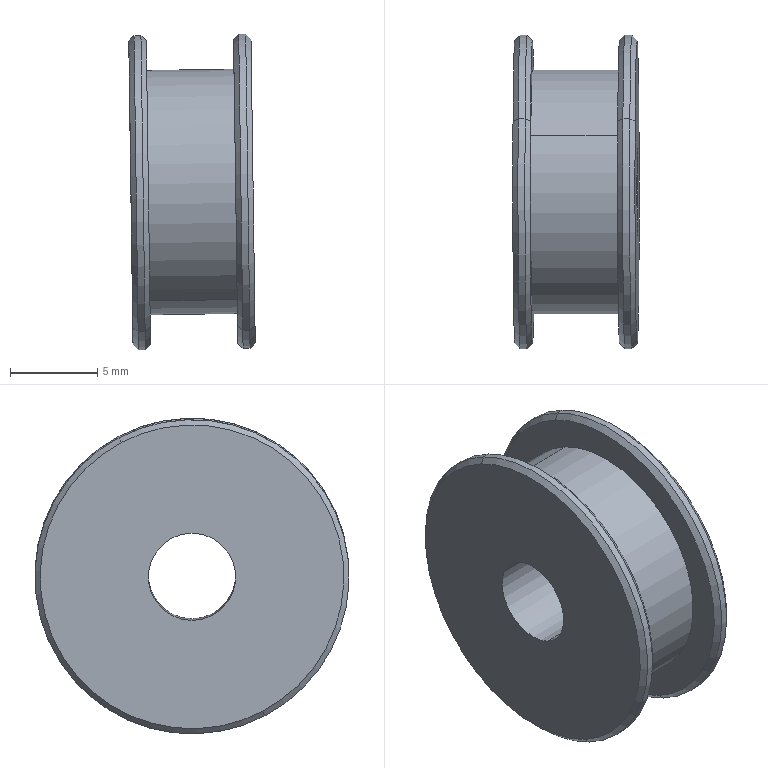Component | SolidWorks | DA-0220-Part11-12 | 1 solid | 20 faces | box 7.24 x 18 x 18.09 mm | volume 1131 mm3 | cone 8 | cylinder 8 | plane 4 | commonest cylinder face diameters 18 x4 14 x2 5 x2
build123d program:
from build123d import *

# Parameters (mm, degrees)
CHAMFER1_SIZE = 0.3


with BuildPart() as part:
    # Sketch1 → Revolve1 (revolve)
    with BuildSketch(Plane.XY, mode=Mode.PRIVATE) as revolve1_sk:
        Polygon((-9, 3.5), (-2.5, 3.5), (-2.5, -3.5), (-9, -3.5), (-9, -2.5), (-7, -2.5), (-7, 2.5), (-9, 2.5), align=None)
    revolve(revolve1_sk.sketch.rotate(Axis((0, 0, 0), (0, -1, 0)), 270), axis=Axis((0, 0, 0), (0, -1, 0)))

    # Chamfer1
    chamfer1_edges = [part.edges().sort_by_distance(p)[0] for p in [
        (0, 2.5, -9),
        (0, -2.5, -9),
        (0, -3.5, -9),
        (0, 3.5, -9),
    ]]
    chamfer(chamfer1_edges, length=CHAMFER1_SIZE)


solid = part.part

# Placed as in the assembly
solid = solid.moved(Location((642.057, -33.791, 552.514), (177.304, 0.7997, 90.014)))
STEP:
#1=COLOUR_RGB('',0.7922,0.8196,0.9333);
#2=FILL_AREA_STYLE_COLOUR('',#1);
#3=FILL_AREA_STYLE('',(#2));
#4=SURFACE_STYLE_FILL_AREA(#3);
#5=SURFACE_SIDE_STYLE('',(#4));
#6=SURFACE_STYLE_USAGE(.BOTH.,#5);
#7=PRESENTATION_STYLE_ASSIGNMENT((#6));
#8=CARTESIAN_POINT('',(25.184,-1.49,21.448));
#9=VERTEX_POINT('',#8);
#10=CARTESIAN_POINT('',(25.175,-1.171,22.054));
#11=VERTEX_POINT('',#10);
#12=CARTESIAN_POINT('',(25.179,-1.33,21.751));
#13=DIRECTION('',(0.9999,0.000404,0.01395));
#14=DIRECTION('',(0.01254,-0.4647,-0.8854));
#15=AXIS2_PLACEMENT_3D('',#12,#13,#14);
#16=CIRCLE('',#15,0.3425);
#17=EDGE_CURVE('',#9,#11,#16,.T.);
#18=ORIENTED_EDGE('',*,*,#17,.F.);
#19=CARTESIAN_POINT('',(25.172,-1.495,21.437));
#20=VERTEX_POINT('',#19);
#21=CARTESIAN_POINT('',(25.172,-1.495,21.437));
#22=DIRECTION('',(-0.6982,-0.3289,-0.6359));
#23=VECTOR('',#22,39.37);
#24=LINE('',#21,#23);
#25=EDGE_CURVE('',#9,#20,#24,.T.);
#26=ORIENTED_EDGE('',*,*,#25,.T.);
#27=CARTESIAN_POINT('',(25.163,-1.166,22.065));
#28=VERTEX_POINT('',#27);
#29=CARTESIAN_POINT('',(25.168,-1.33,21.751));
#30=DIRECTION('',(-0.9999,-0.000404,-0.01395));
#31=DIRECTION('',(0.01254,-0.4647,-0.8854));
#32=AXIS2_PLACEMENT_3D('',#29,#30,#31);
#33=CIRCLE('',#32,0.3543);
#34=EDGE_CURVE('',#28,#20,#33,.T.);
#35=ORIENTED_EDGE('',*,*,#34,.F.);
#36=CARTESIAN_POINT('',(25.163,-1.166,22.065));
#37=DIRECTION('',(-0.7159,0.3283,0.6162));
#38=VECTOR('',#37,39.37);
#39=LINE('',#36,#38);
#40=EDGE_CURVE('',#11,#28,#39,.T.);
#41=ORIENTED_EDGE('',*,*,#40,.F.);
#42=EDGE_LOOP('',(#18,#26,#35,#41));
#43=FACE_OUTER_BOUND('',#42,.T.);
#44=CARTESIAN_POINT('',(25.168,-1.33,21.751));
#45=DIRECTION('',(-0.9999,-0.000404,-0.01395));
#46=DIRECTION('',(-0.01254,0.4647,0.8854));
#47=AXIS2_PLACEMENT_3D('',#44,#45,#46);
#48=CONICAL_SURFACE('',#47,0.3543,0.7854);
#49=ADVANCED_FACE('',(#43),#48,.T.);
#50=CARTESIAN_POINT('',(25.372,-1.171,22.057));
#51=VERTEX_POINT('',#50);
#52=CARTESIAN_POINT('',(25.381,-1.49,21.451));
#53=VERTEX_POINT('',#52);
#54=CARTESIAN_POINT('',(25.376,-1.33,21.754));
#55=DIRECTION('',(-0.9999,-0.000404,-0.01395));
#56=DIRECTION('',(-0.01254,0.4647,0.8854));
#57=AXIS2_PLACEMENT_3D('',#54,#55,#56);
#58=CIRCLE('',#57,0.3425);
#59=EDGE_CURVE('',#51,#53,#58,.T.);
#60=ORIENTED_EDGE('',*,*,#59,.F.);
#61=CARTESIAN_POINT('',(25.384,-1.166,22.068));
#62=VERTEX_POINT('',#61);
#63=CARTESIAN_POINT('',(25.372,-1.171,22.057));
#64=DIRECTION('',(0.6982,0.3289,0.6359));
#65=VECTOR('',#64,39.37);
#66=LINE('',#63,#65);
#67=EDGE_CURVE('',#51,#62,#66,.T.);
#68=ORIENTED_EDGE('',*,*,#67,.T.);
#69=CARTESIAN_POINT('',(25.393,-1.495,21.44));
#70=VERTEX_POINT('',#69);
#71=CARTESIAN_POINT('',(25.388,-1.33,21.754));
#72=DIRECTION('',(0.9999,0.000404,0.01395));
#73=DIRECTION('',(-0.01254,0.4647,0.8854));
#74=AXIS2_PLACEMENT_3D('',#71,#72,#73);
#75=CIRCLE('',#74,0.3543);
#76=EDGE_CURVE('',#70,#62,#75,.T.);
#77=ORIENTED_EDGE('',*,*,#76,.F.);
#78=CARTESIAN_POINT('',(25.381,-1.49,21.451));
#79=DIRECTION('',(0.7159,-0.3283,-0.6162));
#80=VECTOR('',#79,39.37);
#81=LINE('',#78,#80);
#82=EDGE_CURVE('',#53,#70,#81,.T.);
#83=ORIENTED_EDGE('',*,*,#82,.F.);
#84=EDGE_LOOP('',(#60,#68,#77,#83));
#85=FACE_OUTER_BOUND('',#84,.T.);
#86=CARTESIAN_POINT('',(25.376,-1.33,21.754));
#87=DIRECTION('',(0.9999,0.000404,0.01395));
#88=DIRECTION('',(0.01254,-0.4647,-0.8854));
#89=AXIS2_PLACEMENT_3D('',#86,#87,#88);
#90=CONICAL_SURFACE('',#89,0.3425,0.7854);
#91=ADVANCED_FACE('',(#85),#90,.T.);
#92=CARTESIAN_POINT('',(25.42,-1.489,21.451));
#93=VERTEX_POINT('',#92);
#94=CARTESIAN_POINT('',(25.411,-1.171,22.058));
#95=VERTEX_POINT('',#94);
#96=CARTESIAN_POINT('',(25.416,-1.33,21.754));
#97=DIRECTION('',(0.9999,0.000404,0.01395));
#98=DIRECTION('',(0.01254,-0.4647,-0.8854));
#99=AXIS2_PLACEMENT_3D('',#96,#97,#98);
#100=CIRCLE('',#99,0.3425);
#101=EDGE_CURVE('',#93,#95,#100,.T.);
#102=ORIENTED_EDGE('',*,*,#101,.F.);
#103=CARTESIAN_POINT('',(25.408,-1.495,21.441));
#104=VERTEX_POINT('',#103);
#105=CARTESIAN_POINT('',(25.408,-1.495,21.441));
#106=DIRECTION('',(-0.6982,-0.3289,-0.6359));
#107=VECTOR('',#106,39.37);
#108=LINE('',#105,#107);
#109=EDGE_CURVE('',#93,#104,#108,.T.);
#110=ORIENTED_EDGE('',*,*,#109,.T.);
#111=CARTESIAN_POINT('',(25.399,-1.166,22.068));
#112=VERTEX_POINT('',#111);
#113=CARTESIAN_POINT('',(25.404,-1.33,21.754));
#114=DIRECTION('',(-0.9999,-0.000404,-0.01395));
#115=DIRECTION('',(0.01254,-0.4647,-0.8854));
#116=AXIS2_PLACEMENT_3D('',#113,#114,#115);
#117=CIRCLE('',#116,0.3543);
#118=EDGE_CURVE('',#112,#104,#117,.T.);
#119=ORIENTED_EDGE('',*,*,#118,.F.);
#120=CARTESIAN_POINT('',(25.399,-1.166,22.068));
#121=DIRECTION('',(-0.7159,0.3283,0.6162));
#122=VECTOR('',#121,39.37);
#123=LINE('',#120,#122);
#124=EDGE_CURVE('',#95,#112,#123,.T.);
#125=ORIENTED_EDGE('',*,*,#124,.F.);
#126=EDGE_LOOP('',(#102,#110,#119,#125));
#127=FACE_OUTER_BOUND('',#126,.T.);
#128=CARTESIAN_POINT('',(25.404,-1.33,21.754));
#129=DIRECTION('',(-0.9999,-0.000404,-0.01395));
#130=DIRECTION('',(-0.01254,0.4647,0.8854));
#131=AXIS2_PLACEMENT_3D('',#128,#129,#130);
#132=CONICAL_SURFACE('',#131,0.3543,0.7854);
#133=ADVANCED_FACE('',(#127),#132,.T.);
#134=CARTESIAN_POINT('',(25.136,-1.171,22.054));
#135=VERTEX_POINT('',#134);
#136=CARTESIAN_POINT('',(25.144,-1.49,21.447));
#137=VERTEX_POINT('',#136);
#138=CARTESIAN_POINT('',(25.14,-1.33,21.751));
#139=DIRECTION('',(-0.9999,-0.000404,-0.01395));
#140=DIRECTION('',(-0.01254,0.4647,0.8854));
#141=AXIS2_PLACEMENT_3D('',#138,#139,#140);
#142=CIRCLE('',#141,0.3425);
#143=EDGE_CURVE('',#135,#137,#142,.T.);
#144=ORIENTED_EDGE('',*,*,#143,.F.);
#145=CARTESIAN_POINT('',(25.147,-1.166,22.064));
#146=VERTEX_POINT('',#145);
#147=CARTESIAN_POINT('',(25.136,-1.171,22.054));
#148=DIRECTION('',(0.6982,0.3289,0.6359));
#149=VECTOR('',#148,39.37);
#150=LINE('',#147,#149);
#151=EDGE_CURVE('',#135,#146,#150,.T.);
#152=ORIENTED_EDGE('',*,*,#151,.T.);
#153=CARTESIAN_POINT('',(25.156,-1.495,21.437));
#154=VERTEX_POINT('',#153);
#155=CARTESIAN_POINT('',(25.152,-1.33,21.751));
#156=DIRECTION('',(0.9999,0.000404,0.01395));
#157=DIRECTION('',(-0.01254,0.4647,0.8854));
#158=AXIS2_PLACEMENT_3D('',#155,#156,#157);
#159=CIRCLE('',#158,0.3543);
#160=EDGE_CURVE('',#154,#146,#159,.T.);
#161=ORIENTED_EDGE('',*,*,#160,.F.);
#162=CARTESIAN_POINT('',(25.144,-1.49,21.447));
#163=DIRECTION('',(0.7159,-0.3283,-0.6162));
#164=VECTOR('',#163,39.37);
#165=LINE('',#162,#164);
#166=EDGE_CURVE('',#137,#154,#165,.T.);
#167=ORIENTED_EDGE('',*,*,#166,.F.);
#168=EDGE_LOOP('',(#144,#152,#161,#167));
#169=FACE_OUTER_BOUND('',#168,.T.);
#170=CARTESIAN_POINT('',(25.14,-1.33,21.751));
#171=DIRECTION('',(0.9999,0.000404,0.01395));
#172=DIRECTION('',(0.01254,-0.4647,-0.8854));
#173=AXIS2_PLACEMENT_3D('',#170,#171,#172);
#174=CONICAL_SURFACE('',#173,0.3425,0.7854);
#175=ADVANCED_FACE('',(#169),#174,.T.);
#176=CARTESIAN_POINT('',(25.373,-1.202,21.998));
#177=VERTEX_POINT('',#176);
#178=CARTESIAN_POINT('',(25.38,-1.458,21.51));
#179=VERTEX_POINT('',#178);
#180=CARTESIAN_POINT('',(25.376,-1.33,21.754));
#181=DIRECTION('',(-0.9999,-0.000404,-0.01395));
#182=DIRECTION('',(-0.01254,0.4647,0.8854));
#183=AXIS2_PLACEMENT_3D('',#180,#181,#182);
#184=CIRCLE('',#183,0.2756);
#185=EDGE_CURVE('',#177,#179,#184,.T.);
#186=ORIENTED_EDGE('',*,*,#185,.T.);
#187=CARTESIAN_POINT('',(25.183,-1.458,21.507));
#188=VERTEX_POINT('',#187);
#189=CARTESIAN_POINT('',(25.281,-1.458,21.509));
#190=DIRECTION('',(-0.9999,-0.000404,-0.01395));
#191=VECTOR('',#190,39.37);
#192=LINE('',#189,#191);
#193=EDGE_CURVE('',#179,#188,#192,.T.);
#194=ORIENTED_EDGE('',*,*,#193,.T.);
#195=CARTESIAN_POINT('',(25.176,-1.202,21.995));
#196=VERTEX_POINT('',#195);
#197=CARTESIAN_POINT('',(25.179,-1.33,21.751));
#198=DIRECTION('',(-0.9999,-0.000404,-0.01395));
#199=DIRECTION('',(-0.01254,0.4647,0.8854));
#200=AXIS2_PLACEMENT_3D('',#197,#198,#199);
#201=CIRCLE('',#200,0.2756);
#202=EDGE_CURVE('',#196,#188,#201,.T.);
#203=ORIENTED_EDGE('',*,*,#202,.F.);
#204=CARTESIAN_POINT('',(25.274,-1.202,21.997));
#205=DIRECTION('',(-0.9999,-0.000404,-0.01395));
#206=VECTOR('',#205,39.37);
#207=LINE('',#204,#206);
#208=EDGE_CURVE('',#177,#196,#207,.T.);
#209=ORIENTED_EDGE('',*,*,#208,.F.);
#210=EDGE_LOOP('',(#186,#194,#203,#209));
#211=FACE_OUTER_BOUND('',#210,.T.);
#212=CARTESIAN_POINT('',(25.278,-1.33,21.753));
#213=DIRECTION('',(-0.9999,-0.000404,-0.01395));
#214=DIRECTION('',(-0.01254,0.4647,0.8854));
#215=AXIS2_PLACEMENT_3D('',#212,#213,#214);
#216=CYLINDRICAL_SURFACE('',#215,0.2756);
#217=ADVANCED_FACE('',(#211),#216,.T.);
#218=ORIENTED_EDGE('',*,*,#118,.T.);
#219=CARTESIAN_POINT('',(25.282,-1.495,21.439));
#220=DIRECTION('',(-0.9999,-0.000404,-0.01395));
#221=VECTOR('',#220,39.37);
#222=LINE('',#219,#221);
#223=EDGE_CURVE('',#104,#70,#222,.T.);
#224=ORIENTED_EDGE('',*,*,#223,.T.);
#225=ORIENTED_EDGE('',*,*,#76,.T.);
#226=CARTESIAN_POINT('',(25.273,-1.166,22.066));
#227=DIRECTION('',(-0.9999,-0.000404,-0.01395));
#228=VECTOR('',#227,39.37);
#229=LINE('',#226,#228);
#230=EDGE_CURVE('',#112,#62,#229,.T.);
#231=ORIENTED_EDGE('',*,*,#230,.F.);
#232=EDGE_LOOP('',(#218,#224,#225,#231));
#233=FACE_OUTER_BOUND('',#232,.T.);
#234=CARTESIAN_POINT('',(25.278,-1.33,21.753));
#235=DIRECTION('',(-0.9999,-0.000404,-0.01395));
#236=DIRECTION('',(-0.01254,0.4647,0.8854));
#237=AXIS2_PLACEMENT_3D('',#234,#235,#236);
#238=CYLINDRICAL_SURFACE('',#237,0.3543);
#239=ADVANCED_FACE('',(#233),#238,.T.);
#240=CARTESIAN_POINT('',(25.417,-1.376,21.667));
#241=VERTEX_POINT('',#240);
#242=CARTESIAN_POINT('',(25.414,-1.285,21.842));
#243=VERTEX_POINT('',#242);
#244=CARTESIAN_POINT('',(25.416,-1.33,21.754));
#245=DIRECTION('',(-0.9999,-0.000404,-0.01395));
#246=DIRECTION('',(-0.01254,0.4647,0.8854));
#247=AXIS2_PLACEMENT_3D('',#244,#245,#246);
#248=CIRCLE('',#247,0.09843);
#249=EDGE_CURVE('',#241,#243,#248,.T.);
#250=ORIENTED_EDGE('',*,*,#249,.F.);
#251=CARTESIAN_POINT('',(25.141,-1.376,21.663));
#252=VERTEX_POINT('',#251);
#253=CARTESIAN_POINT('',(25.279,-1.376,21.665));
#254=DIRECTION('',(-0.9999,-0.000404,-0.01395));
#255=VECTOR('',#254,39.37);
#256=LINE('',#253,#255);
#257=EDGE_CURVE('',#241,#252,#256,.T.);
#258=ORIENTED_EDGE('',*,*,#257,.T.);
#259=CARTESIAN_POINT('',(25.139,-1.285,21.838));
#260=VERTEX_POINT('',#259);
#261=CARTESIAN_POINT('',(25.14,-1.33,21.751));
#262=DIRECTION('',(-0.9999,-0.000404,-0.01395));
#263=DIRECTION('',(-0.01254,0.4647,0.8854));
#264=AXIS2_PLACEMENT_3D('',#261,#262,#263);
#265=CIRCLE('',#264,0.09843);
#266=EDGE_CURVE('',#252,#260,#265,.T.);
#267=ORIENTED_EDGE('',*,*,#266,.T.);
#268=CARTESIAN_POINT('',(25.277,-1.285,21.84));
#269=DIRECTION('',(-0.9999,-0.000404,-0.01395));
#270=VECTOR('',#269,39.37);
#271=LINE('',#268,#270);
#272=EDGE_CURVE('',#243,#260,#271,.T.);
#273=ORIENTED_EDGE('',*,*,#272,.F.);
#274=EDGE_LOOP('',(#250,#258,#267,#273));
#275=FACE_OUTER_BOUND('',#274,.T.);
#276=CARTESIAN_POINT('',(25.278,-1.33,21.753));
#277=DIRECTION('',(-0.9999,-0.000404,-0.01395));
#278=DIRECTION('',(-0.01254,0.4647,0.8854));
#279=AXIS2_PLACEMENT_3D('',#276,#277,#278);
#280=CYLINDRICAL_SURFACE('',#279,0.09843);
#281=ADVANCED_FACE('',(#275),#280,.F.);
#282=ORIENTED_EDGE('',*,*,#34,.T.);
#283=CARTESIAN_POINT('',(25.282,-1.495,21.439));
#284=DIRECTION('',(-0.9999,-0.000404,-0.01395));
#285=VECTOR('',#284,39.37);
#286=LINE('',#283,#285);
#287=EDGE_CURVE('',#20,#154,#286,.T.);
#288=ORIENTED_EDGE('',*,*,#287,.T.);
#289=ORIENTED_EDGE('',*,*,#160,.T.);
#290=CARTESIAN_POINT('',(25.273,-1.166,22.066));
#291=DIRECTION('',(-0.9999,-0.000404,-0.01395));
#292=VECTOR('',#291,39.37);
#293=LINE('',#290,#292);
#294=EDGE_CURVE('',#28,#146,#293,.T.);
#295=ORIENTED_EDGE('',*,*,#294,.F.);
#296=EDGE_LOOP('',(#282,#288,#289,#295));
#297=FACE_OUTER_BOUND('',#296,.T.);
#298=CARTESIAN_POINT('',(25.278,-1.33,21.753));
#299=DIRECTION('',(-0.9999,-0.000404,-0.01395));
#300=DIRECTION('',(-0.01254,0.4647,0.8854));
#301=AXIS2_PLACEMENT_3D('',#298,#299,#300);
#302=CYLINDRICAL_SURFACE('',#301,0.3543);
#303=ADVANCED_FACE('',(#297),#302,.T.);
#304=ORIENTED_EDGE('',*,*,#287,.F.);
#305=CARTESIAN_POINT('',(25.168,-1.33,21.751));
#306=DIRECTION('',(-0.9999,-0.000404,-0.01395));
#307=DIRECTION('',(0.01254,-0.4647,-0.8854));
#308=AXIS2_PLACEMENT_3D('',#305,#306,#307);
#309=CIRCLE('',#308,0.3543);
#310=EDGE_CURVE('',#20,#28,#309,.T.);
#311=ORIENTED_EDGE('',*,*,#310,.T.);
#312=ORIENTED_EDGE('',*,*,#294,.T.);
#313=CARTESIAN_POINT('',(25.152,-1.33,21.751));
#314=DIRECTION('',(0.9999,0.000404,0.01395));
#315=DIRECTION('',(-0.01254,0.4647,0.8854));
#316=AXIS2_PLACEMENT_3D('',#313,#314,#315);
#317=CIRCLE('',#316,0.3543);
#318=EDGE_CURVE('',#146,#154,#317,.T.);
#319=ORIENTED_EDGE('',*,*,#318,.T.);
#320=EDGE_LOOP('',(#304,#311,#312,#319));
#321=FACE_OUTER_BOUND('',#320,.T.);
#322=CARTESIAN_POINT('',(25.278,-1.33,21.753));
#323=DIRECTION('',(-0.9999,-0.000404,-0.01395));
#324=DIRECTION('',(-0.01254,0.4647,0.8854));
#325=AXIS2_PLACEMENT_3D('',#322,#323,#324);
#326=CYLINDRICAL_SURFACE('',#325,0.3543);
#327=ADVANCED_FACE('',(#321),#326,.T.);
#328=CARTESIAN_POINT('',(25.14,-1.33,21.751));
#329=DIRECTION('',(-0.9999,-0.000404,-0.01395));
#330=DIRECTION('',(-0.01254,0.4647,0.8854));
#331=AXIS2_PLACEMENT_3D('',#328,#329,#330);
#332=CIRCLE('',#331,0.3425);
#333=EDGE_CURVE('',#137,#135,#332,.T.);
#334=ORIENTED_EDGE('',*,*,#333,.T.);
#335=ORIENTED_EDGE('',*,*,#143,.T.);
#336=EDGE_LOOP('',(#334,#335));
#337=FACE_OUTER_BOUND('',#336,.T.);
#338=CARTESIAN_POINT('',(25.14,-1.33,21.751));
#339=DIRECTION('',(-0.9999,-0.000404,-0.01395));
#340=DIRECTION('',(-0.01254,0.4647,0.8854));
#341=AXIS2_PLACEMENT_3D('',#338,#339,#340);
#342=CIRCLE('',#341,0.09843);
#343=EDGE_CURVE('',#260,#252,#342,.T.);
#344=ORIENTED_EDGE('',*,*,#343,.F.);
#345=ORIENTED_EDGE('',*,*,#266,.F.);
#346=EDGE_LOOP('',(#344,#345));
#347=FACE_BOUND('',#346,.T.);
#348=CARTESIAN_POINT('',(25.138,-1.644,21.915));
#349=DIRECTION('',(-0.9999,-0.000404,-0.01395));
#350=DIRECTION('',(-0.01254,0.4647,0.8854));
#351=AXIS2_PLACEMENT_3D('',#348,#349,#350);
#352=PLANE('',#351);
#353=ADVANCED_FACE('',(#337,#347),#352,.T.);
#354=ORIENTED_EDGE('',*,*,#257,.F.);
#355=CARTESIAN_POINT('',(25.416,-1.33,21.754));
#356=DIRECTION('',(-0.9999,-0.000404,-0.01395));
#357=DIRECTION('',(-0.01254,0.4647,0.8854));
#358=AXIS2_PLACEMENT_3D('',#355,#356,#357);
#359=CIRCLE('',#358,0.09843);
#360=EDGE_CURVE('',#243,#241,#359,.T.);
#361=ORIENTED_EDGE('',*,*,#360,.F.);
#362=ORIENTED_EDGE('',*,*,#272,.T.);
#363=ORIENTED_EDGE('',*,*,#343,.T.);
#364=EDGE_LOOP('',(#354,#361,#362,#363));
#365=FACE_OUTER_BOUND('',#364,.T.);
#366=CARTESIAN_POINT('',(25.278,-1.33,21.753));
#367=DIRECTION('',(-0.9999,-0.000404,-0.01395));
#368=DIRECTION('',(-0.01254,0.4647,0.8854));
#369=AXIS2_PLACEMENT_3D('',#366,#367,#368);
#370=CYLINDRICAL_SURFACE('',#369,0.09843);
#371=ADVANCED_FACE('',(#365),#370,.F.);
#372=CARTESIAN_POINT('',(25.416,-1.33,21.754));
#373=DIRECTION('',(0.9999,0.000404,0.01395));
#374=DIRECTION('',(0.01254,-0.4647,-0.8854));
#375=AXIS2_PLACEMENT_3D('',#372,#373,#374);
#376=CIRCLE('',#375,0.3425);
#377=EDGE_CURVE('',#95,#93,#376,.T.);
#378=ORIENTED_EDGE('',*,*,#377,.T.);
#379=ORIENTED_EDGE('',*,*,#101,.T.);
#380=EDGE_LOOP('',(#378,#379));
#381=FACE_OUTER_BOUND('',#380,.T.);
#382=ORIENTED_EDGE('',*,*,#360,.T.);
#383=ORIENTED_EDGE('',*,*,#249,.T.);
#384=EDGE_LOOP('',(#382,#383));
#385=FACE_BOUND('',#384,.T.);
#386=CARTESIAN_POINT('',(25.415,-1.417,21.8));
#387=DIRECTION('',(0.9999,0.000404,0.01395));
#388=DIRECTION('',(0.01254,-0.4647,-0.8854));
#389=AXIS2_PLACEMENT_3D('',#386,#387,#388);
#390=PLANE('',#389);
#391=ADVANCED_FACE('',(#381,#385),#390,.T.);
#392=ORIENTED_EDGE('',*,*,#223,.F.);
#393=CARTESIAN_POINT('',(25.404,-1.33,21.754));
#394=DIRECTION('',(-0.9999,-0.000404,-0.01395));
#395=DIRECTION('',(0.01254,-0.4647,-0.8854));
#396=AXIS2_PLACEMENT_3D('',#393,#394,#395);
#397=CIRCLE('',#396,0.3543);
#398=EDGE_CURVE('',#104,#112,#397,.T.);
#399=ORIENTED_EDGE('',*,*,#398,.T.);
#400=ORIENTED_EDGE('',*,*,#230,.T.);
#401=CARTESIAN_POINT('',(25.388,-1.33,21.754));
#402=DIRECTION('',(0.9999,0.000404,0.01395));
#403=DIRECTION('',(-0.01254,0.4647,0.8854));
#404=AXIS2_PLACEMENT_3D('',#401,#402,#403);
#405=CIRCLE('',#404,0.3543);
#406=EDGE_CURVE('',#62,#70,#405,.T.);
#407=ORIENTED_EDGE('',*,*,#406,.T.);
#408=EDGE_LOOP('',(#392,#399,#400,#407));
#409=FACE_OUTER_BOUND('',#408,.T.);
#410=CARTESIAN_POINT('',(25.278,-1.33,21.753));
#411=DIRECTION('',(-0.9999,-0.000404,-0.01395));
#412=DIRECTION('',(-0.01254,0.4647,0.8854));
#413=AXIS2_PLACEMENT_3D('',#410,#411,#412);
#414=CYLINDRICAL_SURFACE('',#413,0.3543);
#415=ADVANCED_FACE('',(#409),#414,.T.);
#416=CARTESIAN_POINT('',(25.376,-1.33,21.754));
#417=DIRECTION('',(-0.9999,-0.000404,-0.01395));
#418=DIRECTION('',(-0.01254,0.4647,0.8854));
#419=AXIS2_PLACEMENT_3D('',#416,#417,#418);
#420=CIRCLE('',#419,0.3425);
#421=EDGE_CURVE('',#53,#51,#420,.T.);
#422=ORIENTED_EDGE('',*,*,#421,.T.);
#423=ORIENTED_EDGE('',*,*,#59,.T.);
#424=EDGE_LOOP('',(#422,#423));
#425=FACE_OUTER_BOUND('',#424,.T.);
#426=ORIENTED_EDGE('',*,*,#185,.F.);
#427=CARTESIAN_POINT('',(25.376,-1.33,21.754));
#428=DIRECTION('',(-0.9999,-0.000404,-0.01395));
#429=DIRECTION('',(-0.01254,0.4647,0.8854));
#430=AXIS2_PLACEMENT_3D('',#427,#428,#429);
#431=CIRCLE('',#430,0.2756);
#432=EDGE_CURVE('',#179,#177,#431,.T.);
#433=ORIENTED_EDGE('',*,*,#432,.F.);
#434=EDGE_LOOP('',(#426,#433));
#435=FACE_BOUND('',#434,.T.);
#436=CARTESIAN_POINT('',(25.374,-1.644,21.919));
#437=DIRECTION('',(-0.9999,-0.000404,-0.01395));
#438=DIRECTION('',(-0.01254,0.4647,0.8854));
#439=AXIS2_PLACEMENT_3D('',#436,#437,#438);
#440=PLANE('',#439);
#441=ADVANCED_FACE('',(#425,#435),#440,.T.);
#442=ORIENTED_EDGE('',*,*,#193,.F.);
#443=ORIENTED_EDGE('',*,*,#432,.T.);
#444=ORIENTED_EDGE('',*,*,#208,.T.);
#445=CARTESIAN_POINT('',(25.179,-1.33,21.751));
#446=DIRECTION('',(-0.9999,-0.000404,-0.01395));
#447=DIRECTION('',(-0.01254,0.4647,0.8854));
#448=AXIS2_PLACEMENT_3D('',#445,#446,#447);
#449=CIRCLE('',#448,0.2756);
#450=EDGE_CURVE('',#188,#196,#449,.T.);
#451=ORIENTED_EDGE('',*,*,#450,.F.);
#452=EDGE_LOOP('',(#442,#443,#444,#451));
#453=FACE_OUTER_BOUND('',#452,.T.);
#454=CARTESIAN_POINT('',(25.278,-1.33,21.753));
#455=DIRECTION('',(-0.9999,-0.000404,-0.01395));
#456=DIRECTION('',(-0.01254,0.4647,0.8854));
#457=AXIS2_PLACEMENT_3D('',#454,#455,#456);
#458=CYLINDRICAL_SURFACE('',#457,0.2756);
#459=ADVANCED_FACE('',(#453),#458,.T.);
#460=CARTESIAN_POINT('',(25.179,-1.33,21.751));
#461=DIRECTION('',(0.9999,0.000404,0.01395));
#462=DIRECTION('',(0.01254,-0.4647,-0.8854));
#463=AXIS2_PLACEMENT_3D('',#460,#461,#462);
#464=CIRCLE('',#463,0.3425);
#465=EDGE_CURVE('',#11,#9,#464,.T.);
#466=ORIENTED_EDGE('',*,*,#465,.T.);
#467=ORIENTED_EDGE('',*,*,#17,.T.);
#468=EDGE_LOOP('',(#466,#467));
#469=FACE_OUTER_BOUND('',#468,.T.);
#470=ORIENTED_EDGE('',*,*,#202,.T.);
#471=ORIENTED_EDGE('',*,*,#450,.T.);
#472=EDGE_LOOP('',(#470,#471));
#473=FACE_BOUND('',#472,.T.);
#474=CARTESIAN_POINT('',(25.178,-1.574,21.879));
#475=DIRECTION('',(0.9999,0.000404,0.01395));
#476=DIRECTION('',(0.01254,-0.4647,-0.8854));
#477=AXIS2_PLACEMENT_3D('',#474,#475,#476);
#478=PLANE('',#477);
#479=ADVANCED_FACE('',(#469,#473),#478,.T.);
#480=ORIENTED_EDGE('',*,*,#151,.F.);
#481=ORIENTED_EDGE('',*,*,#333,.F.);
#482=ORIENTED_EDGE('',*,*,#166,.T.);
#483=ORIENTED_EDGE('',*,*,#318,.F.);
#484=EDGE_LOOP('',(#480,#481,#482,#483));
#485=FACE_OUTER_BOUND('',#484,.T.);
#486=CARTESIAN_POINT('',(25.14,-1.33,21.751));
#487=DIRECTION('',(0.9999,0.000404,0.01395));
#488=DIRECTION('',(0.01254,-0.4647,-0.8854));
#489=AXIS2_PLACEMENT_3D('',#486,#487,#488);
#490=CONICAL_SURFACE('',#489,0.3425,0.7854);
#491=ADVANCED_FACE('',(#485),#490,.T.);
#492=ORIENTED_EDGE('',*,*,#109,.F.);
#493=ORIENTED_EDGE('',*,*,#377,.F.);
#494=ORIENTED_EDGE('',*,*,#124,.T.);
#495=ORIENTED_EDGE('',*,*,#398,.F.);
#496=EDGE_LOOP('',(#492,#493,#494,#495));
#497=FACE_OUTER_BOUND('',#496,.T.);
#498=CARTESIAN_POINT('',(25.404,-1.33,21.754));
#499=DIRECTION('',(-0.9999,-0.000404,-0.01395));
#500=DIRECTION('',(-0.01254,0.4647,0.8854));
#501=AXIS2_PLACEMENT_3D('',#498,#499,#500);
#502=CONICAL_SURFACE('',#501,0.3543,0.7854);
#503=ADVANCED_FACE('',(#497),#502,.T.);
#504=ORIENTED_EDGE('',*,*,#67,.F.);
#505=ORIENTED_EDGE('',*,*,#421,.F.);
#506=ORIENTED_EDGE('',*,*,#82,.T.);
#507=ORIENTED_EDGE('',*,*,#406,.F.);
#508=EDGE_LOOP('',(#504,#505,#506,#507));
#509=FACE_OUTER_BOUND('',#508,.T.);
#510=CARTESIAN_POINT('',(25.376,-1.33,21.754));
#511=DIRECTION('',(0.9999,0.000404,0.01395));
#512=DIRECTION('',(0.01254,-0.4647,-0.8854));
#513=AXIS2_PLACEMENT_3D('',#510,#511,#512);
#514=CONICAL_SURFACE('',#513,0.3425,0.7854);
#515=ADVANCED_FACE('',(#509),#514,.T.);
#516=ORIENTED_EDGE('',*,*,#25,.F.);
#517=ORIENTED_EDGE('',*,*,#465,.F.);
#518=ORIENTED_EDGE('',*,*,#40,.T.);
#519=ORIENTED_EDGE('',*,*,#310,.F.);
#520=EDGE_LOOP('',(#516,#517,#518,#519));
#521=FACE_OUTER_BOUND('',#520,.T.);
#522=CARTESIAN_POINT('',(25.168,-1.33,21.751));
#523=DIRECTION('',(-0.9999,-0.000404,-0.01395));
#524=DIRECTION('',(-0.01254,0.4647,0.8854));
#525=AXIS2_PLACEMENT_3D('',#522,#523,#524);
#526=CONICAL_SURFACE('',#525,0.3543,0.7854);
#527=ADVANCED_FACE('',(#521),#526,.T.);
#528=CLOSED_SHELL('',(#49,#91,#133,#175,#217,#239,#281,#303,#327,#353,#371,#391,#415,#441,#459,#479,#491,#503,#515,#527));
#529=MANIFOLD_SOLID_BREP('',#528);
#530=STYLED_ITEM('',(#7),#529);
#531=PRESENTATION_LAYER_ASSIGNMENT('','',(#530));
#532=(LENGTH_UNIT()NAMED_UNIT(*)SI_UNIT($,.METRE.));
#533=LENGTH_MEASURE_WITH_UNIT(LENGTH_MEASURE(0.0254),#532);
#534=DIMENSIONAL_EXPONENTS(1.,0.,0.,0.,0.,0.,0.);
#535=(CONVERSION_BASED_UNIT('',#533)LENGTH_UNIT()NAMED_UNIT(#534));
#536=UNCERTAINTY_MEASURE_WITH_UNIT(LENGTH_MEASURE(0.00001),#535,'','');
#537=(NAMED_UNIT(*)PLANE_ANGLE_UNIT()SI_UNIT($,.RADIAN.));
#538=(NAMED_UNIT(*)SI_UNIT($,.STERADIAN.)SOLID_ANGLE_UNIT());
#539=(GEOMETRIC_REPRESENTATION_CONTEXT(3)GLOBAL_UNCERTAINTY_ASSIGNED_CONTEXT((#536))GLOBAL_UNIT_ASSIGNED_CONTEXT((#535,#537,#538))REPRESENTATION_CONTEXT('',''));
#540=MECHANICAL_DESIGN_GEOMETRIC_PRESENTATION_REPRESENTATION('',(#530),#539);
#541=CARTESIAN_POINT('',(0.,0.,0.));
#542=DIRECTION('',(0.,0.,1.));
#543=DIRECTION('',(1.,0.,0.));
#544=AXIS2_PLACEMENT_3D('',#541,#542,#543);
#545=(LENGTH_UNIT()NAMED_UNIT(*)SI_UNIT($,.METRE.));
#546=LENGTH_MEASURE_WITH_UNIT(LENGTH_MEASURE(0.0254),#545);
#547=DIMENSIONAL_EXPONENTS(1.,0.,0.,0.,0.,0.,0.);
#548=(CONVERSION_BASED_UNIT('',#546)LENGTH_UNIT()NAMED_UNIT(#547));
#549=UNCERTAINTY_MEASURE_WITH_UNIT(LENGTH_MEASURE(0.00001),#548,'','');
#550=(NAMED_UNIT(*)PLANE_ANGLE_UNIT()SI_UNIT($,.RADIAN.));
#551=(NAMED_UNIT(*)SI_UNIT($,.STERADIAN.)SOLID_ANGLE_UNIT());
#552=(GEOMETRIC_REPRESENTATION_CONTEXT(3)GLOBAL_UNCERTAINTY_ASSIGNED_CONTEXT((#549))GLOBAL_UNIT_ASSIGNED_CONTEXT((#548,#550,#551))REPRESENTATION_CONTEXT('',''));
#553=ADVANCED_BREP_SHAPE_REPRESENTATION('',(#529,#544),#552);